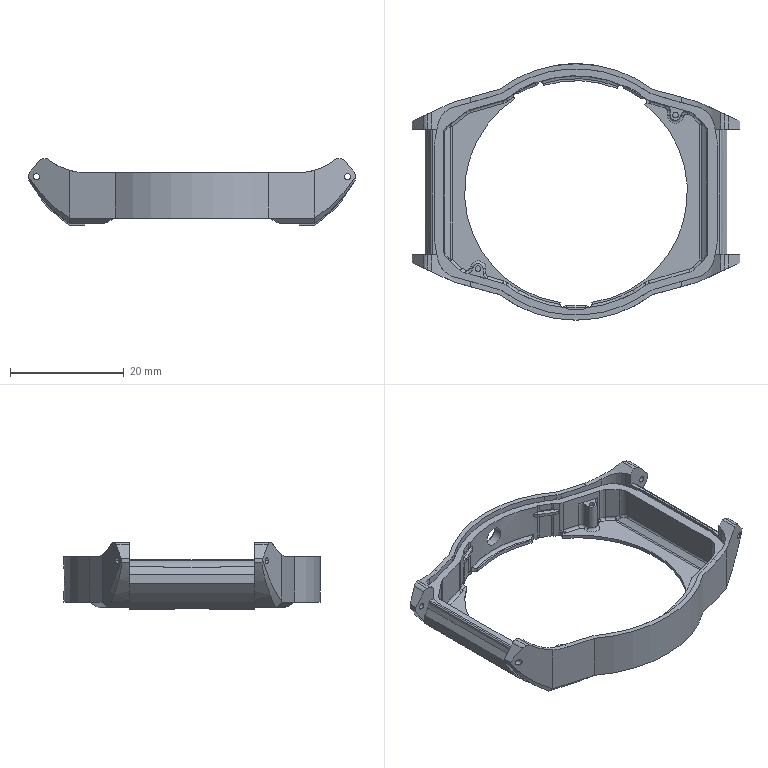CAM job | NX | mm | 3-axis | 1 set-up | 2 operations | part box 57.5 x 45 x 11.75
set-up 1
1. Cavity Milling | Mill Mill5 T1 | CAVITY_MILL | path 41891.115 mm | 81.055 min
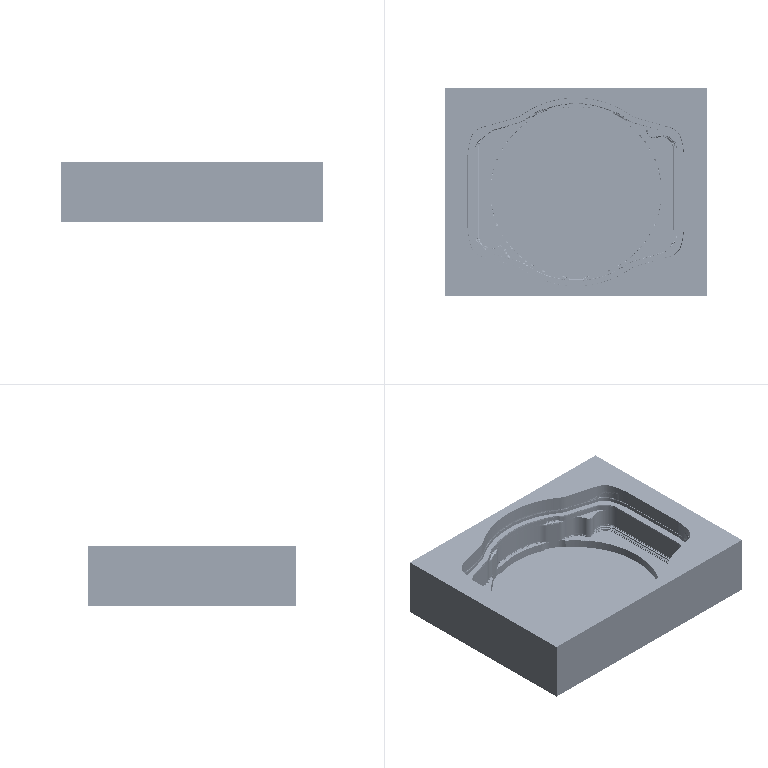2. Cavity Milling | Mill Mill5 T2 | CAVITY_MILL_COPY | path 22280.442 mm | 42.542 min